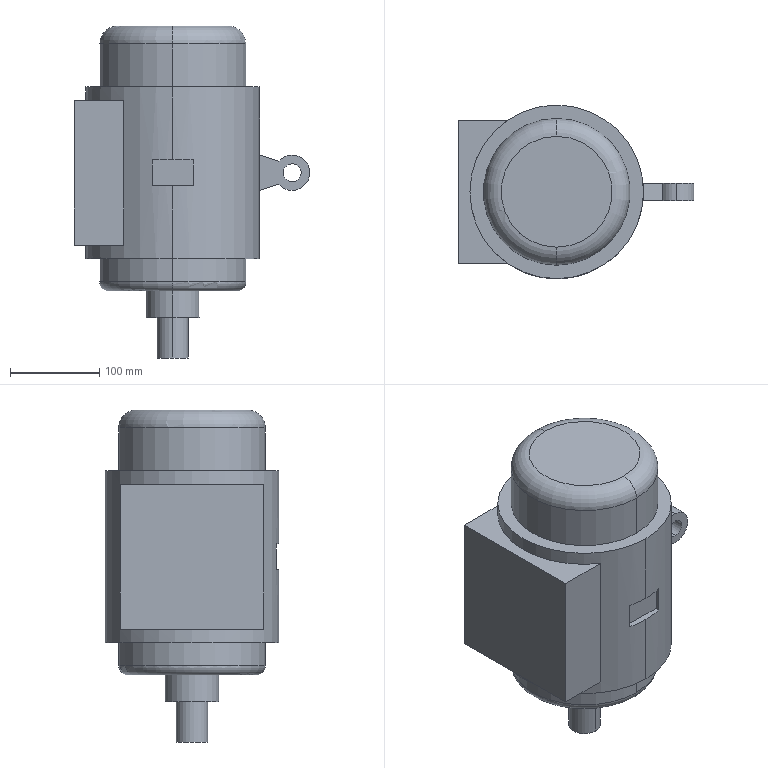Component | SolidWorks | Motor-1 | 2 solids | 40 faces | box 263.22 x 194 x 371 mm | volume 8632529 mm3 | plane 21 | cylinder 15 | torus 4 | commonest cylinder face diameters 164 x4 39.478 x3 20 x2 35 x2 60 x2 194 x2
build123d program:
from build123d import *

# Parameters (mm, degrees)
SKETCH1_R           = 97
BOSS_EXTRUDE1_DEPTH = 192
SKETCH2_R           = 82
BOSS_EXTRUDE2_DEPTH = 68
FILLET1_R           = 20
BOSS_EXTRUDE3_START = 36
SKETCH3_R           = 82
BOSS_EXTRUDE3_DEPTH = 36
FILLET2_R           = 10
SKETCH4_R           = 30
BOSS_EXTRUDE4_DEPTH = 30
SKETCH5_R           = 17.5
BOSS_EXTRUDE5_DEPTH = 45
SKETCH6_W           = 162
SKETCH6_H           = 160
BOSS_EXTRUDE6_DEPTH = 65
SKETCH7_R           = 10
BOSS_EXTRUDE7_DEPTH = 20
SKETCH8_W           = 28.856
SKETCH8_H           = 46.031
CUT_EXTRUDE1_DEPTH  = 10


with BuildPart() as part:
    # Sketch1 → Boss-Extrude1 (new body)
    with BuildSketch(Plane(origin=(0, 0, 0), x_dir=(0, 0, -1), z_dir=(1, 0, 0))):
        Circle(SKETCH1_R)
    extrude(amount=BOSS_EXTRUDE1_DEPTH)

    # Sketch2 → Boss-Extrude2 (add)
    with BuildSketch(Plane(origin=(192, 0, 0), x_dir=(0, 0, -1), z_dir=(1, 0, 0))):
        Circle(SKETCH2_R)
    extrude(amount=BOSS_EXTRUDE2_DEPTH)

    # Fillet1
    fillet1_edges = [part.edges().sort_by_distance(p)[0] for p in [
        (260, 0, 82),
    ]]
    fillet(fillet1_edges, radius=FILLET1_R)

    # Sketch3 → Boss-Extrude3 (add)
    with BuildSketch(Plane.ZY.offset(BOSS_EXTRUDE3_START)):
        with Locations(Location((0, 0, 0), (0, 0, 180))):
            Circle(SKETCH3_R)
    extrude(amount=-BOSS_EXTRUDE3_DEPTH)

    # Fillet2
    fillet2_edges = [part.edges().sort_by_distance(p)[0] for p in [
        (-36, 0, 82),
    ]]
    fillet(fillet2_edges, radius=FILLET2_R)

    # Sketch4 → Boss-Extrude4 (add)
    with BuildSketch(Plane.ZY.offset(36)):
        Circle(SKETCH4_R)
    extrude(amount=BOSS_EXTRUDE4_DEPTH)

    # Sketch5 → Boss-Extrude5 (add)
    with BuildSketch(Plane.ZY.offset(66)):
        with Locations(Location((0, 0, 0), (0, 0, 180))):
            Circle(SKETCH5_R)
    extrude(amount=BOSS_EXTRUDE5_DEPTH)

    # Sketch6 → Boss-Extrude6 (add)
    with BuildSketch(Plane(origin=(0, 110, 0), x_dir=(1, 0, 0), z_dir=(0, 1, 0))):
        with Locations((96, 0)):
            Rectangle(SKETCH6_W, SKETCH6_H)
    extrude(amount=-BOSS_EXTRUDE6_DEPTH)

    # Sketch8 → Cut-Extrude1 (cut)
    with BuildSketch(Plane.XY.offset(100)):
        with Locations((96, 0)):
            Rectangle(SKETCH8_W, SKETCH8_H)
    extrude(amount=-CUT_EXTRUDE1_DEPTH, mode=Mode.SUBTRACT)


with BuildPart() as body_2:
    # Sketch7 → Boss-Extrude7 (new body)
    with BuildSketch(Plane.XY.offset(10)):
        with BuildLine():
            Line((116, -97), (76, -97))
            Line((76, -97), (83.169, -118.485))
            ThreePointArc((83.169, -118.485), (96, -153.224), (108.831, -118.485))
            Line((108.831, -118.485), (116, -97))
        make_face()
        with Locations((96, -133.485)):
            Circle(SKETCH7_R, mode=Mode.SUBTRACT)
    extrude(amount=-BOSS_EXTRUDE7_DEPTH)


solid = Compound([part.part, body_2.part])

# Placed as in the assembly
solid = solid.moved(Location((549.733, 15.31, 211.072), (90, 0, 90)))